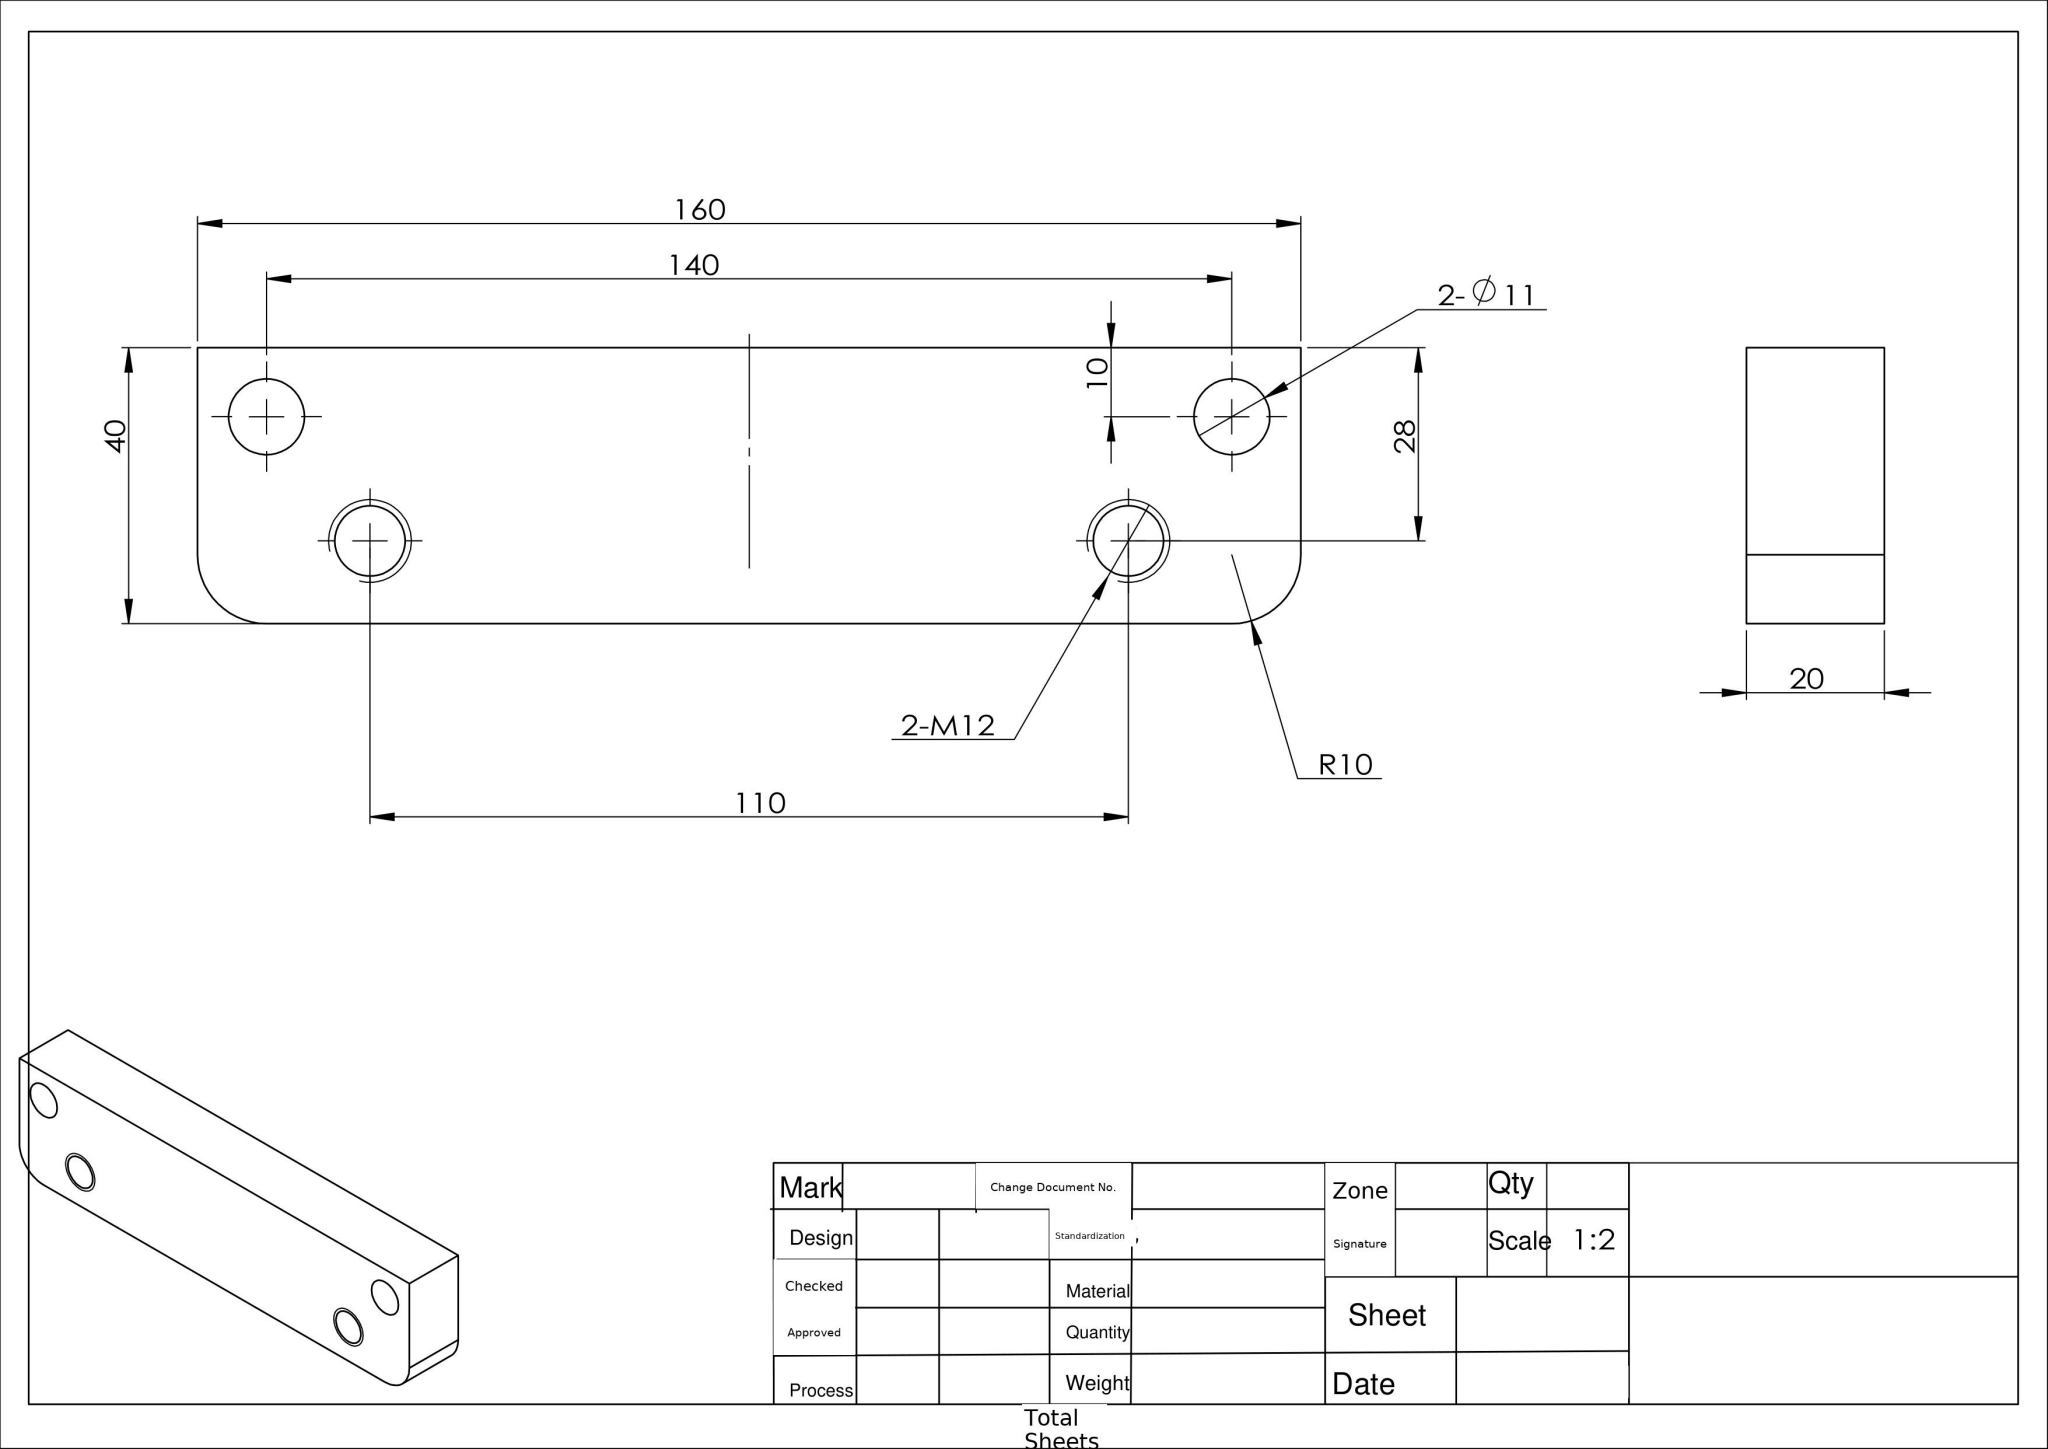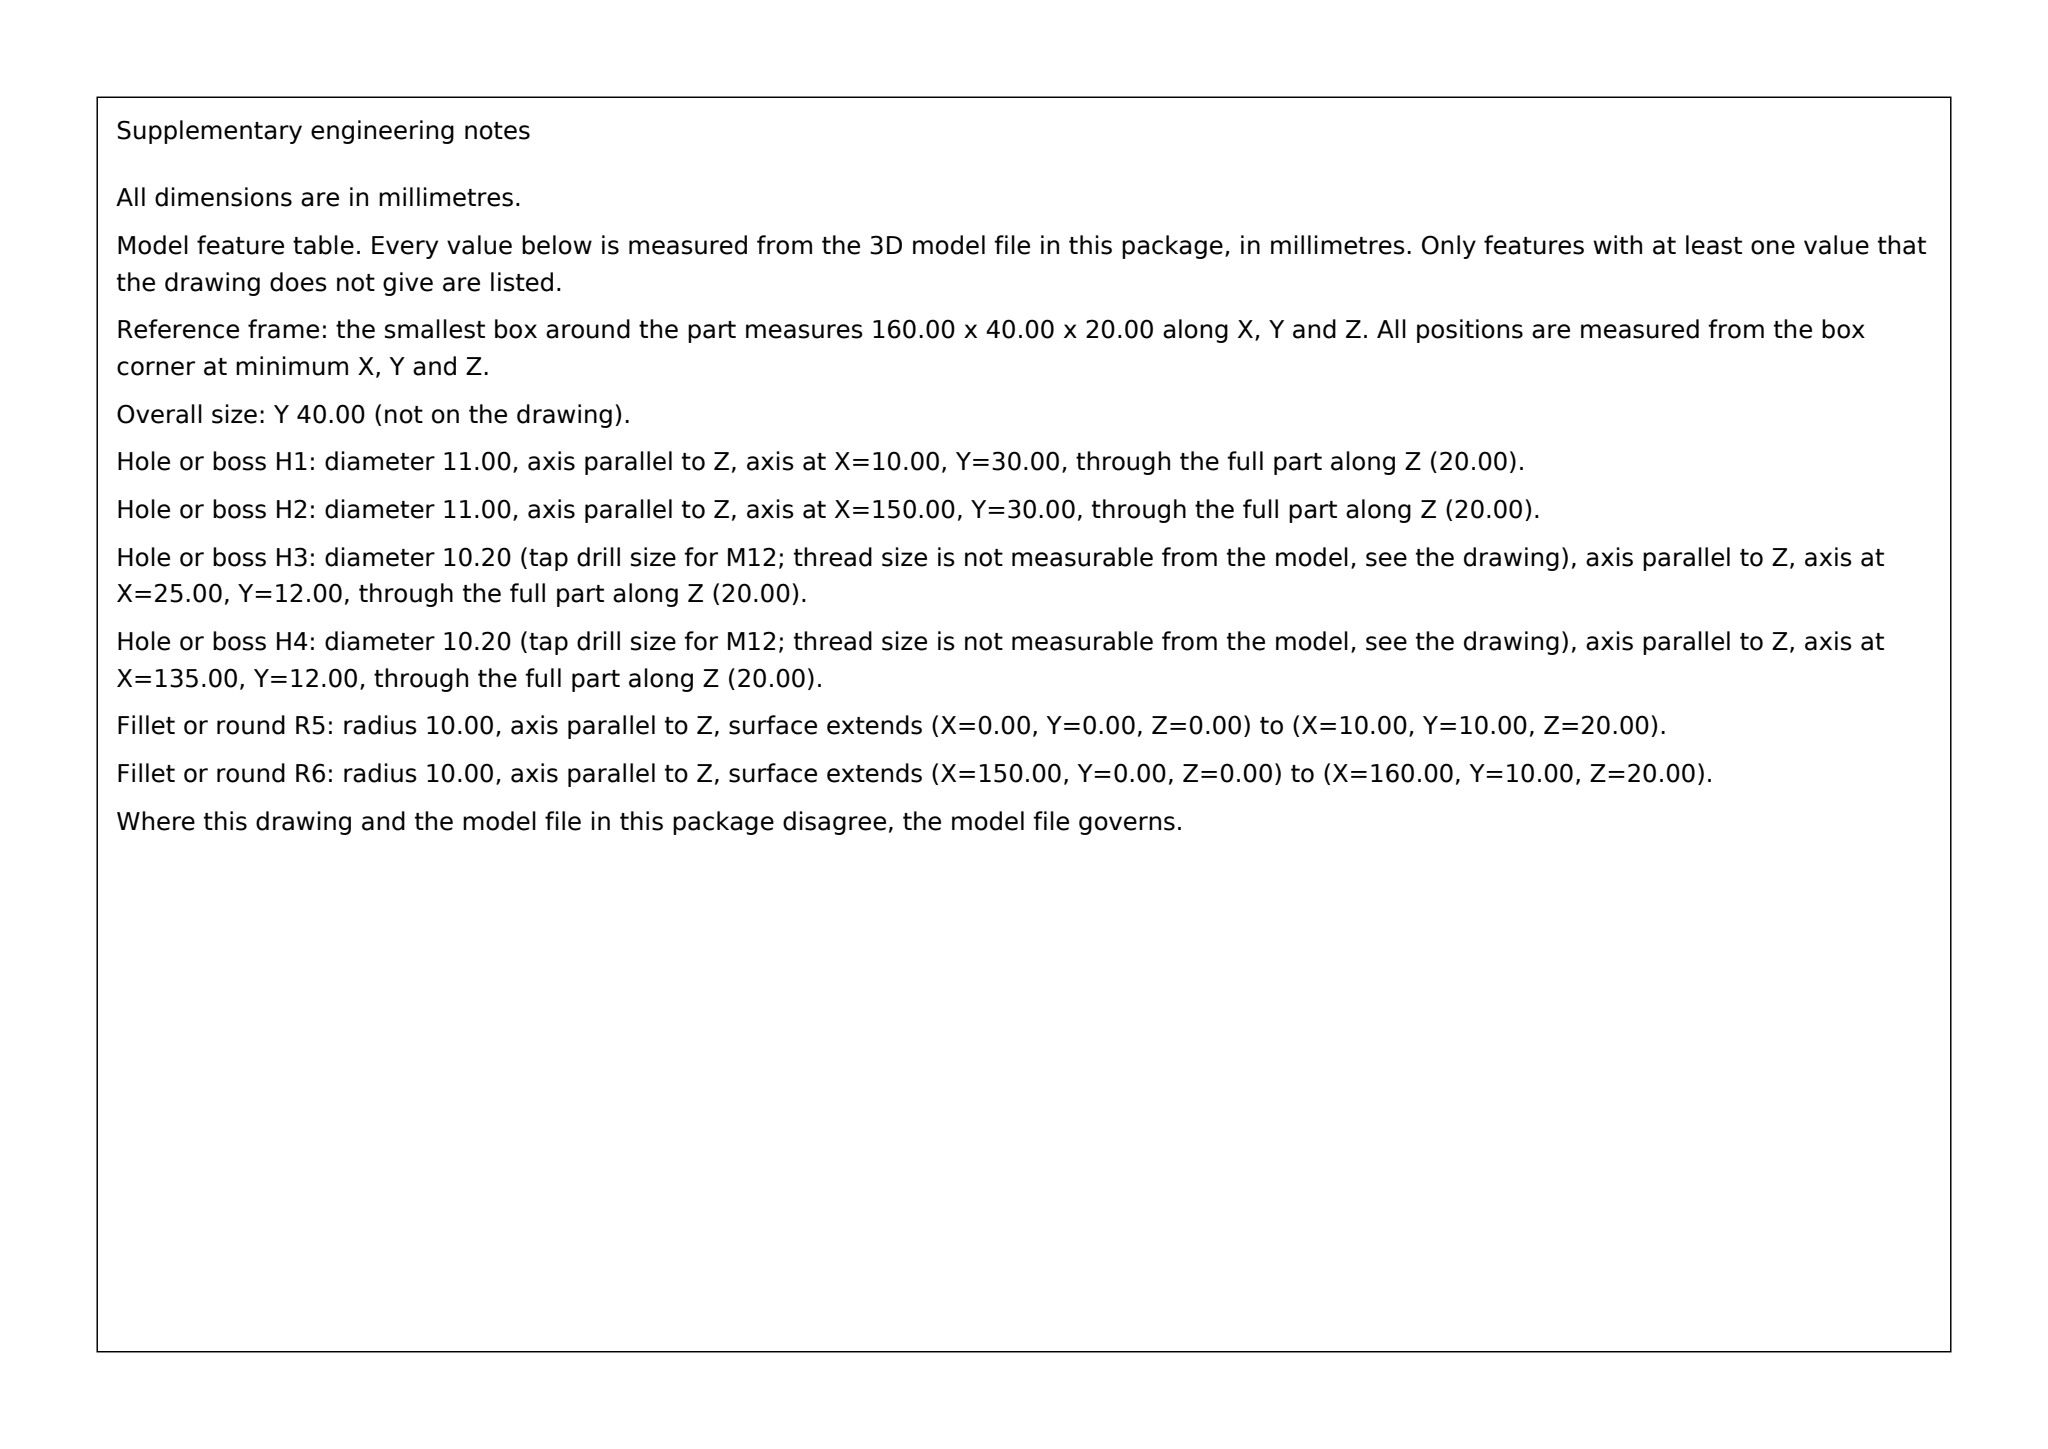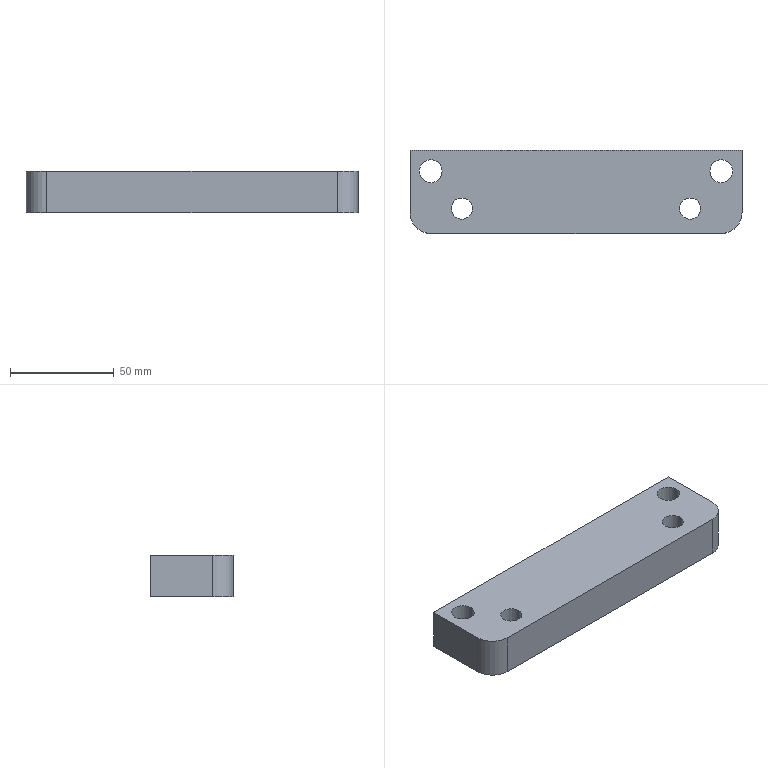Part | SolidWorks | 1 solid | 16 faces | box 160 x 40 x 20 mm | volume 120072 mm3 | cylinder 10 | plane 6 | commonest cylinder face diameters 10.2 x4 11 x4 20 x2
build123d program:
from build123d import *

# Parameters (mm, degrees)
SKETCH1_W              = 160
SKETCH1_H              = 40
BOSS_EXTRUDE1_DEPTH    = 20
SKETCH2_R              = 5.5
CUT_EXTRUDE1_DEPTH     = 20
M12_TAPPED_HOLE1_D     = 10.2
M12_TAPPED_HOLE1_DEPTH = 32.75
M12_TAPPED_HOLE1_TIP   = 3.064
FILLET1_R              = 10


with BuildPart() as part:
    # Sketch1 → Boss-Extrude1 (new body)
    with BuildSketch(Plane.XY):
        with Locations((80, 20)):
            Rectangle(SKETCH1_W, SKETCH1_H)
    extrude(amount=BOSS_EXTRUDE1_DEPTH)

    # Sketch2 → Cut-Extrude1 (cut)
    with BuildSketch(Plane.XY.offset(20)):
        with Locations((10, 30)):
            Circle(SKETCH2_R)
        with Locations((150, 30)):
            Circle(SKETCH2_R)
    extrude(amount=-CUT_EXTRUDE1_DEPTH, mode=Mode.SUBTRACT)

    # M12 Tapped Hole1
    with Locations(Plane.XY.offset(20)):
        with Locations((25, 12), (135, 12)):
            Hole(M12_TAPPED_HOLE1_D / 2, depth=M12_TAPPED_HOLE1_DEPTH)
            with Locations((0, 0, -(M12_TAPPED_HOLE1_DEPTH + M12_TAPPED_HOLE1_TIP / 2))):  # 118° drill point
                Cone(0, M12_TAPPED_HOLE1_D / 2, M12_TAPPED_HOLE1_TIP, mode=Mode.SUBTRACT)

    # Fillet1
    fillet1_edges = [part.edges().sort_by_distance(p)[0] for p in [
        (160, 0, 10),
        (0, 0, 10),
    ]]
    fillet(fillet1_edges, radius=FILLET1_R)


solid = part.part
STEP:
#1=CARTESIAN_POINT('',(30.1,12.,0.));
#2=VERTEX_POINT('',#1);
#3=CARTESIAN_POINT('',(19.9,12.,0.));
#4=VERTEX_POINT('',#3);
#5=CARTESIAN_POINT('',(25.,12.,0.));
#6=DIRECTION('',(0.,0.,-1.));
#7=DIRECTION('',(-1.,0.,0.));
#8=AXIS2_PLACEMENT_3D('',#5,#6,#7);
#9=CIRCLE('',#8,5.1);
#10=EDGE_CURVE('',#2,#4,#9,.T.);
#11=ORIENTED_EDGE('',*,*,#10,.T.);
#12=CARTESIAN_POINT('',(19.9,12.,20.));
#13=VERTEX_POINT('',#12);
#14=CARTESIAN_POINT('',(19.9,12.,20.));
#15=DIRECTION('',(0.,0.,1.));
#16=VECTOR('',#15,1000.);
#17=LINE('',#14,#16);
#18=EDGE_CURVE('',#4,#13,#17,.T.);
#19=ORIENTED_EDGE('',*,*,#18,.T.);
#20=CARTESIAN_POINT('',(30.1,12.,20.));
#21=VERTEX_POINT('',#20);
#22=CARTESIAN_POINT('',(25.,12.,20.));
#23=DIRECTION('',(0.,0.,1.));
#24=DIRECTION('',(1.,0.,0.));
#25=AXIS2_PLACEMENT_3D('',#22,#23,#24);
#26=CIRCLE('',#25,5.1);
#27=EDGE_CURVE('',#13,#21,#26,.T.);
#28=ORIENTED_EDGE('',*,*,#27,.T.);
#29=CARTESIAN_POINT('',(30.1,12.,20.));
#30=DIRECTION('',(0.,0.,1.));
#31=VECTOR('',#30,1000.);
#32=LINE('',#29,#31);
#33=EDGE_CURVE('',#2,#21,#32,.T.);
#34=ORIENTED_EDGE('',*,*,#33,.F.);
#35=EDGE_LOOP('',(#11,#19,#28,#34));
#36=FACE_OUTER_BOUND('',#35,.T.);
#37=CARTESIAN_POINT('',(25.,12.,20.));
#38=DIRECTION('',(0.,0.,1.));
#39=DIRECTION('',(1.,0.,0.));
#40=AXIS2_PLACEMENT_3D('',#37,#38,#39);
#41=CYLINDRICAL_SURFACE('',#40,5.1);
#42=ADVANCED_FACE('',(#36),#41,.F.);
#43=CARTESIAN_POINT('',(140.1,12.,0.));
#44=VERTEX_POINT('',#43);
#45=CARTESIAN_POINT('',(129.9,12.,0.));
#46=VERTEX_POINT('',#45);
#47=CARTESIAN_POINT('',(135.,12.,0.));
#48=DIRECTION('',(0.,0.,-1.));
#49=DIRECTION('',(-1.,0.,0.));
#50=AXIS2_PLACEMENT_3D('',#47,#48,#49);
#51=CIRCLE('',#50,5.1);
#52=EDGE_CURVE('',#44,#46,#51,.T.);
#53=ORIENTED_EDGE('',*,*,#52,.T.);
#54=CARTESIAN_POINT('',(129.9,12.,20.));
#55=VERTEX_POINT('',#54);
#56=CARTESIAN_POINT('',(129.9,12.,20.));
#57=DIRECTION('',(0.,0.,1.));
#58=VECTOR('',#57,1000.);
#59=LINE('',#56,#58);
#60=EDGE_CURVE('',#46,#55,#59,.T.);
#61=ORIENTED_EDGE('',*,*,#60,.T.);
#62=CARTESIAN_POINT('',(140.1,12.,20.));
#63=VERTEX_POINT('',#62);
#64=CARTESIAN_POINT('',(135.,12.,20.));
#65=DIRECTION('',(0.,0.,1.));
#66=DIRECTION('',(1.,0.,0.));
#67=AXIS2_PLACEMENT_3D('',#64,#65,#66);
#68=CIRCLE('',#67,5.1);
#69=EDGE_CURVE('',#55,#63,#68,.T.);
#70=ORIENTED_EDGE('',*,*,#69,.T.);
#71=CARTESIAN_POINT('',(140.1,12.,20.));
#72=DIRECTION('',(0.,0.,1.));
#73=VECTOR('',#72,1000.);
#74=LINE('',#71,#73);
#75=EDGE_CURVE('',#44,#63,#74,.T.);
#76=ORIENTED_EDGE('',*,*,#75,.F.);
#77=EDGE_LOOP('',(#53,#61,#70,#76));
#78=FACE_OUTER_BOUND('',#77,.T.);
#79=CARTESIAN_POINT('',(135.,12.,20.));
#80=DIRECTION('',(0.,0.,1.));
#81=DIRECTION('',(1.,0.,0.));
#82=AXIS2_PLACEMENT_3D('',#79,#80,#81);
#83=CYLINDRICAL_SURFACE('',#82,5.1);
#84=ADVANCED_FACE('',(#78),#83,.F.);
#85=CARTESIAN_POINT('',(144.5,30.,0.));
#86=VERTEX_POINT('',#85);
#87=CARTESIAN_POINT('',(155.5,30.,0.));
#88=VERTEX_POINT('',#87);
#89=CARTESIAN_POINT('',(150.,30.,0.));
#90=DIRECTION('',(0.,0.,1.));
#91=DIRECTION('',(1.,0.,0.));
#92=AXIS2_PLACEMENT_3D('',#89,#90,#91);
#93=CIRCLE('',#92,5.5);
#94=EDGE_CURVE('',#86,#88,#93,.T.);
#95=ORIENTED_EDGE('',*,*,#94,.F.);
#96=CARTESIAN_POINT('',(144.5,30.,20.));
#97=VERTEX_POINT('',#96);
#98=CARTESIAN_POINT('',(144.5,30.,0.));
#99=DIRECTION('',(0.,0.,1.));
#100=VECTOR('',#99,1000.);
#101=LINE('',#98,#100);
#102=EDGE_CURVE('',#86,#97,#101,.T.);
#103=ORIENTED_EDGE('',*,*,#102,.T.);
#104=CARTESIAN_POINT('',(155.5,30.,20.));
#105=VERTEX_POINT('',#104);
#106=CARTESIAN_POINT('',(150.,30.,20.));
#107=DIRECTION('',(0.,0.,1.));
#108=DIRECTION('',(1.,0.,0.));
#109=AXIS2_PLACEMENT_3D('',#106,#107,#108);
#110=CIRCLE('',#109,5.5);
#111=EDGE_CURVE('',#97,#105,#110,.T.);
#112=ORIENTED_EDGE('',*,*,#111,.T.);
#113=CARTESIAN_POINT('',(155.5,30.,0.));
#114=DIRECTION('',(0.,0.,1.));
#115=VECTOR('',#114,1000.);
#116=LINE('',#113,#115);
#117=EDGE_CURVE('',#88,#105,#116,.T.);
#118=ORIENTED_EDGE('',*,*,#117,.F.);
#119=EDGE_LOOP('',(#95,#103,#112,#118));
#120=FACE_OUTER_BOUND('',#119,.T.);
#121=CARTESIAN_POINT('',(150.,30.,0.));
#122=DIRECTION('',(0.,0.,1.));
#123=DIRECTION('',(1.,0.,0.));
#124=AXIS2_PLACEMENT_3D('',#121,#122,#123);
#125=CYLINDRICAL_SURFACE('',#124,5.5);
#126=ADVANCED_FACE('',(#120),#125,.F.);
#127=CARTESIAN_POINT('',(4.5,30.,0.));
#128=VERTEX_POINT('',#127);
#129=CARTESIAN_POINT('',(15.5,30.,0.));
#130=VERTEX_POINT('',#129);
#131=CARTESIAN_POINT('',(10.,30.,0.));
#132=DIRECTION('',(0.,0.,1.));
#133=DIRECTION('',(1.,0.,0.));
#134=AXIS2_PLACEMENT_3D('',#131,#132,#133);
#135=CIRCLE('',#134,5.5);
#136=EDGE_CURVE('',#128,#130,#135,.T.);
#137=ORIENTED_EDGE('',*,*,#136,.F.);
#138=CARTESIAN_POINT('',(4.5,30.,20.));
#139=VERTEX_POINT('',#138);
#140=CARTESIAN_POINT('',(4.5,30.,0.));
#141=DIRECTION('',(0.,0.,1.));
#142=VECTOR('',#141,1000.);
#143=LINE('',#140,#142);
#144=EDGE_CURVE('',#128,#139,#143,.T.);
#145=ORIENTED_EDGE('',*,*,#144,.T.);
#146=CARTESIAN_POINT('',(15.5,30.,20.));
#147=VERTEX_POINT('',#146);
#148=CARTESIAN_POINT('',(10.,30.,20.));
#149=DIRECTION('',(0.,0.,1.));
#150=DIRECTION('',(1.,0.,0.));
#151=AXIS2_PLACEMENT_3D('',#148,#149,#150);
#152=CIRCLE('',#151,5.5);
#153=EDGE_CURVE('',#139,#147,#152,.T.);
#154=ORIENTED_EDGE('',*,*,#153,.T.);
#155=CARTESIAN_POINT('',(15.5,30.,0.));
#156=DIRECTION('',(0.,0.,1.));
#157=VECTOR('',#156,1000.);
#158=LINE('',#155,#157);
#159=EDGE_CURVE('',#130,#147,#158,.T.);
#160=ORIENTED_EDGE('',*,*,#159,.F.);
#161=EDGE_LOOP('',(#137,#145,#154,#160));
#162=FACE_OUTER_BOUND('',#161,.T.);
#163=CARTESIAN_POINT('',(10.,30.,0.));
#164=DIRECTION('',(0.,0.,1.));
#165=DIRECTION('',(1.,0.,0.));
#166=AXIS2_PLACEMENT_3D('',#163,#164,#165);
#167=CYLINDRICAL_SURFACE('',#166,5.5);
#168=ADVANCED_FACE('',(#162),#167,.F.);
#169=CARTESIAN_POINT('',(0.,40.,0.));
#170=VERTEX_POINT('',#169);
#171=CARTESIAN_POINT('',(0.,10.,0.));
#172=VERTEX_POINT('',#171);
#173=CARTESIAN_POINT('',(0.,0.,0.));
#174=DIRECTION('',(0.,-1.,0.));
#175=VECTOR('',#174,1000.);
#176=LINE('',#173,#175);
#177=EDGE_CURVE('',#170,#172,#176,.T.);
#178=ORIENTED_EDGE('',*,*,#177,.T.);
#179=CARTESIAN_POINT('',(0.,10.,20.));
#180=VERTEX_POINT('',#179);
#181=CARTESIAN_POINT('',(0.,10.,20.));
#182=DIRECTION('',(0.,0.,1.));
#183=VECTOR('',#182,1000.);
#184=LINE('',#181,#183);
#185=EDGE_CURVE('',#172,#180,#184,.T.);
#186=ORIENTED_EDGE('',*,*,#185,.T.);
#187=CARTESIAN_POINT('',(0.,40.,20.));
#188=VERTEX_POINT('',#187);
#189=CARTESIAN_POINT('',(0.,0.,20.));
#190=DIRECTION('',(0.,-1.,0.));
#191=VECTOR('',#190,1000.);
#192=LINE('',#189,#191);
#193=EDGE_CURVE('',#188,#180,#192,.T.);
#194=ORIENTED_EDGE('',*,*,#193,.F.);
#195=CARTESIAN_POINT('',(0.,40.,20.));
#196=DIRECTION('',(0.,0.,-1.));
#197=VECTOR('',#196,1000.);
#198=LINE('',#195,#197);
#199=EDGE_CURVE('',#188,#170,#198,.T.);
#200=ORIENTED_EDGE('',*,*,#199,.T.);
#201=EDGE_LOOP('',(#178,#186,#194,#200));
#202=FACE_OUTER_BOUND('',#201,.T.);
#203=CARTESIAN_POINT('',(0.,0.,20.));
#204=DIRECTION('',(1.,0.,0.));
#205=DIRECTION('',(0.,0.,-1.));
#206=AXIS2_PLACEMENT_3D('',#203,#204,#205);
#207=PLANE('',#206);
#208=ADVANCED_FACE('',(#202),#207,.F.);
#209=CARTESIAN_POINT('',(10.,0.,20.));
#210=VERTEX_POINT('',#209);
#211=CARTESIAN_POINT('',(150.,0.,20.));
#212=VERTEX_POINT('',#211);
#213=CARTESIAN_POINT('',(0.,0.,20.));
#214=DIRECTION('',(1.,0.,0.));
#215=VECTOR('',#214,1000.);
#216=LINE('',#213,#215);
#217=EDGE_CURVE('',#210,#212,#216,.T.);
#218=ORIENTED_EDGE('',*,*,#217,.F.);
#219=CARTESIAN_POINT('',(10.,0.,0.));
#220=VERTEX_POINT('',#219);
#221=CARTESIAN_POINT('',(10.,0.,20.));
#222=DIRECTION('',(0.,0.,-1.));
#223=VECTOR('',#222,1000.);
#224=LINE('',#221,#223);
#225=EDGE_CURVE('',#210,#220,#224,.T.);
#226=ORIENTED_EDGE('',*,*,#225,.T.);
#227=CARTESIAN_POINT('',(150.,0.,0.));
#228=VERTEX_POINT('',#227);
#229=CARTESIAN_POINT('',(0.,0.,0.));
#230=DIRECTION('',(1.,0.,0.));
#231=VECTOR('',#230,1000.);
#232=LINE('',#229,#231);
#233=EDGE_CURVE('',#220,#228,#232,.T.);
#234=ORIENTED_EDGE('',*,*,#233,.T.);
#235=CARTESIAN_POINT('',(150.,0.,20.));
#236=DIRECTION('',(0.,0.,1.));
#237=VECTOR('',#236,1000.);
#238=LINE('',#235,#237);
#239=EDGE_CURVE('',#228,#212,#238,.T.);
#240=ORIENTED_EDGE('',*,*,#239,.T.);
#241=EDGE_LOOP('',(#218,#226,#234,#240));
#242=FACE_OUTER_BOUND('',#241,.T.);
#243=CARTESIAN_POINT('',(0.,0.,20.));
#244=DIRECTION('',(0.,1.,0.));
#245=DIRECTION('',(0.,0.,1.));
#246=AXIS2_PLACEMENT_3D('',#243,#244,#245);
#247=PLANE('',#246);
#248=ADVANCED_FACE('',(#242),#247,.F.);
#249=CARTESIAN_POINT('',(160.,10.,20.));
#250=VERTEX_POINT('',#249);
#251=CARTESIAN_POINT('',(160.,40.,20.));
#252=VERTEX_POINT('',#251);
#253=CARTESIAN_POINT('',(160.,0.,20.));
#254=DIRECTION('',(0.,1.,0.));
#255=VECTOR('',#254,1000.);
#256=LINE('',#253,#255);
#257=EDGE_CURVE('',#250,#252,#256,.T.);
#258=ORIENTED_EDGE('',*,*,#257,.F.);
#259=CARTESIAN_POINT('',(160.,10.,0.));
#260=VERTEX_POINT('',#259);
#261=CARTESIAN_POINT('',(160.,10.,20.));
#262=DIRECTION('',(0.,0.,-1.));
#263=VECTOR('',#262,1000.);
#264=LINE('',#261,#263);
#265=EDGE_CURVE('',#250,#260,#264,.T.);
#266=ORIENTED_EDGE('',*,*,#265,.T.);
#267=CARTESIAN_POINT('',(160.,40.,0.));
#268=VERTEX_POINT('',#267);
#269=CARTESIAN_POINT('',(160.,0.,0.));
#270=DIRECTION('',(0.,1.,0.));
#271=VECTOR('',#270,1000.);
#272=LINE('',#269,#271);
#273=EDGE_CURVE('',#260,#268,#272,.T.);
#274=ORIENTED_EDGE('',*,*,#273,.T.);
#275=CARTESIAN_POINT('',(160.,40.,20.));
#276=DIRECTION('',(0.,0.,-1.));
#277=VECTOR('',#276,1000.);
#278=LINE('',#275,#277);
#279=EDGE_CURVE('',#252,#268,#278,.T.);
#280=ORIENTED_EDGE('',*,*,#279,.F.);
#281=EDGE_LOOP('',(#258,#266,#274,#280));
#282=FACE_OUTER_BOUND('',#281,.T.);
#283=CARTESIAN_POINT('',(160.,0.,20.));
#284=DIRECTION('',(-1.,0.,0.));
#285=DIRECTION('',(0.,0.,1.));
#286=AXIS2_PLACEMENT_3D('',#283,#284,#285);
#287=PLANE('',#286);
#288=ADVANCED_FACE('',(#282),#287,.F.);
#289=CARTESIAN_POINT('',(0.,40.,0.));
#290=DIRECTION('',(-1.,0.,0.));
#291=VECTOR('',#290,1000.);
#292=LINE('',#289,#291);
#293=EDGE_CURVE('',#268,#170,#292,.T.);
#294=ORIENTED_EDGE('',*,*,#293,.T.);
#295=ORIENTED_EDGE('',*,*,#199,.F.);
#296=CARTESIAN_POINT('',(0.,40.,20.));
#297=DIRECTION('',(-1.,0.,0.));
#298=VECTOR('',#297,1000.);
#299=LINE('',#296,#298);
#300=EDGE_CURVE('',#252,#188,#299,.T.);
#301=ORIENTED_EDGE('',*,*,#300,.F.);
#302=ORIENTED_EDGE('',*,*,#279,.T.);
#303=EDGE_LOOP('',(#294,#295,#301,#302));
#304=FACE_OUTER_BOUND('',#303,.T.);
#305=CARTESIAN_POINT('',(0.,40.,20.));
#306=DIRECTION('',(0.,-1.,0.));
#307=DIRECTION('',(0.,0.,-1.));
#308=AXIS2_PLACEMENT_3D('',#305,#306,#307);
#309=PLANE('',#308);
#310=ADVANCED_FACE('',(#304),#309,.F.);
#311=CARTESIAN_POINT('',(25.,12.,20.));
#312=DIRECTION('',(0.,0.,1.));
#313=DIRECTION('',(1.,0.,0.));
#314=AXIS2_PLACEMENT_3D('',#311,#312,#313);
#315=CIRCLE('',#314,5.1);
#316=EDGE_CURVE('',#21,#13,#315,.T.);
#317=ORIENTED_EDGE('',*,*,#316,.F.);
#318=ORIENTED_EDGE('',*,*,#27,.F.);
#319=EDGE_LOOP('',(#317,#318));
#320=FACE_BOUND('',#319,.T.);
#321=CARTESIAN_POINT('',(135.,12.,20.));
#322=DIRECTION('',(0.,0.,1.));
#323=DIRECTION('',(1.,0.,0.));
#324=AXIS2_PLACEMENT_3D('',#321,#322,#323);
#325=CIRCLE('',#324,5.1);
#326=EDGE_CURVE('',#63,#55,#325,.T.);
#327=ORIENTED_EDGE('',*,*,#326,.F.);
#328=ORIENTED_EDGE('',*,*,#69,.F.);
#329=EDGE_LOOP('',(#327,#328));
#330=FACE_BOUND('',#329,.T.);
#331=CARTESIAN_POINT('',(150.,30.,20.));
#332=DIRECTION('',(0.,0.,1.));
#333=DIRECTION('',(1.,0.,0.));
#334=AXIS2_PLACEMENT_3D('',#331,#332,#333);
#335=CIRCLE('',#334,5.5);
#336=EDGE_CURVE('',#105,#97,#335,.T.);
#337=ORIENTED_EDGE('',*,*,#336,.F.);
#338=ORIENTED_EDGE('',*,*,#111,.F.);
#339=EDGE_LOOP('',(#337,#338));
#340=FACE_BOUND('',#339,.T.);
#341=CARTESIAN_POINT('',(10.,30.,20.));
#342=DIRECTION('',(0.,0.,1.));
#343=DIRECTION('',(1.,0.,0.));
#344=AXIS2_PLACEMENT_3D('',#341,#342,#343);
#345=CIRCLE('',#344,5.5);
#346=EDGE_CURVE('',#147,#139,#345,.T.);
#347=ORIENTED_EDGE('',*,*,#346,.F.);
#348=ORIENTED_EDGE('',*,*,#153,.F.);
#349=EDGE_LOOP('',(#347,#348));
#350=FACE_BOUND('',#349,.T.);
#351=ORIENTED_EDGE('',*,*,#193,.T.);
#352=CARTESIAN_POINT('',(10.,10.,20.));
#353=DIRECTION('',(0.,0.,1.));
#354=DIRECTION('',(-1.,0.,0.));
#355=AXIS2_PLACEMENT_3D('',#352,#353,#354);
#356=CIRCLE('',#355,10.);
#357=EDGE_CURVE('',#180,#210,#356,.T.);
#358=ORIENTED_EDGE('',*,*,#357,.T.);
#359=ORIENTED_EDGE('',*,*,#217,.T.);
#360=CARTESIAN_POINT('',(150.,10.,20.));
#361=DIRECTION('',(0.,0.,1.));
#362=DIRECTION('',(-1.,0.,0.));
#363=AXIS2_PLACEMENT_3D('',#360,#361,#362);
#364=CIRCLE('',#363,10.);
#365=EDGE_CURVE('',#212,#250,#364,.T.);
#366=ORIENTED_EDGE('',*,*,#365,.T.);
#367=ORIENTED_EDGE('',*,*,#257,.T.);
#368=ORIENTED_EDGE('',*,*,#300,.T.);
#369=EDGE_LOOP('',(#351,#358,#359,#366,#367,#368));
#370=FACE_OUTER_BOUND('',#369,.T.);
#371=CARTESIAN_POINT('',(0.,0.,20.));
#372=DIRECTION('',(0.,0.,-1.));
#373=DIRECTION('',(-1.,0.,0.));
#374=AXIS2_PLACEMENT_3D('',#371,#372,#373);
#375=PLANE('',#374);
#376=ADVANCED_FACE('',(#320,#330,#340,#350,#370),#375,.F.);
#377=ORIENTED_EDGE('',*,*,#10,.F.);
#378=CARTESIAN_POINT('',(25.,12.,0.));
#379=DIRECTION('',(0.,0.,-1.));
#380=DIRECTION('',(-1.,0.,0.));
#381=AXIS2_PLACEMENT_3D('',#378,#379,#380);
#382=CIRCLE('',#381,5.1);
#383=EDGE_CURVE('',#4,#2,#382,.T.);
#384=ORIENTED_EDGE('',*,*,#383,.F.);
#385=EDGE_LOOP('',(#377,#384));
#386=FACE_BOUND('',#385,.T.);
#387=ORIENTED_EDGE('',*,*,#52,.F.);
#388=CARTESIAN_POINT('',(135.,12.,0.));
#389=DIRECTION('',(0.,0.,-1.));
#390=DIRECTION('',(-1.,0.,0.));
#391=AXIS2_PLACEMENT_3D('',#388,#389,#390);
#392=CIRCLE('',#391,5.1);
#393=EDGE_CURVE('',#46,#44,#392,.T.);
#394=ORIENTED_EDGE('',*,*,#393,.F.);
#395=EDGE_LOOP('',(#387,#394));
#396=FACE_BOUND('',#395,.T.);
#397=CARTESIAN_POINT('',(150.,30.,0.));
#398=DIRECTION('',(0.,0.,1.));
#399=DIRECTION('',(1.,0.,0.));
#400=AXIS2_PLACEMENT_3D('',#397,#398,#399);
#401=CIRCLE('',#400,5.5);
#402=EDGE_CURVE('',#88,#86,#401,.T.);
#403=ORIENTED_EDGE('',*,*,#402,.T.);
#404=ORIENTED_EDGE('',*,*,#94,.T.);
#405=EDGE_LOOP('',(#403,#404));
#406=FACE_BOUND('',#405,.T.);
#407=CARTESIAN_POINT('',(10.,30.,0.));
#408=DIRECTION('',(0.,0.,1.));
#409=DIRECTION('',(1.,0.,0.));
#410=AXIS2_PLACEMENT_3D('',#407,#408,#409);
#411=CIRCLE('',#410,5.5);
#412=EDGE_CURVE('',#130,#128,#411,.T.);
#413=ORIENTED_EDGE('',*,*,#412,.T.);
#414=ORIENTED_EDGE('',*,*,#136,.T.);
#415=EDGE_LOOP('',(#413,#414));
#416=FACE_BOUND('',#415,.T.);
#417=ORIENTED_EDGE('',*,*,#233,.F.);
#418=CARTESIAN_POINT('',(10.,10.,0.));
#419=DIRECTION('',(0.,0.,-1.));
#420=DIRECTION('',(-1.,0.,0.));
#421=AXIS2_PLACEMENT_3D('',#418,#419,#420);
#422=CIRCLE('',#421,10.);
#423=EDGE_CURVE('',#220,#172,#422,.T.);
#424=ORIENTED_EDGE('',*,*,#423,.T.);
#425=ORIENTED_EDGE('',*,*,#177,.F.);
#426=ORIENTED_EDGE('',*,*,#293,.F.);
#427=ORIENTED_EDGE('',*,*,#273,.F.);
#428=CARTESIAN_POINT('',(150.,10.,0.));
#429=DIRECTION('',(0.,0.,-1.));
#430=DIRECTION('',(-1.,0.,0.));
#431=AXIS2_PLACEMENT_3D('',#428,#429,#430);
#432=CIRCLE('',#431,10.);
#433=EDGE_CURVE('',#260,#228,#432,.T.);
#434=ORIENTED_EDGE('',*,*,#433,.T.);
#435=EDGE_LOOP('',(#417,#424,#425,#426,#427,#434));
#436=FACE_OUTER_BOUND('',#435,.T.);
#437=CARTESIAN_POINT('',(0.,0.,0.));
#438=DIRECTION('',(0.,0.,-1.));
#439=DIRECTION('',(-1.,0.,0.));
#440=AXIS2_PLACEMENT_3D('',#437,#438,#439);
#441=PLANE('',#440);
#442=ADVANCED_FACE('',(#386,#396,#406,#416,#436),#441,.T.);
#443=ORIENTED_EDGE('',*,*,#144,.F.);
#444=ORIENTED_EDGE('',*,*,#412,.F.);
#445=ORIENTED_EDGE('',*,*,#159,.T.);
#446=ORIENTED_EDGE('',*,*,#346,.T.);
#447=EDGE_LOOP('',(#443,#444,#445,#446));
#448=FACE_OUTER_BOUND('',#447,.T.);
#449=CARTESIAN_POINT('',(10.,30.,0.));
#450=DIRECTION('',(0.,0.,1.));
#451=DIRECTION('',(1.,0.,0.));
#452=AXIS2_PLACEMENT_3D('',#449,#450,#451);
#453=CYLINDRICAL_SURFACE('',#452,5.5);
#454=ADVANCED_FACE('',(#448),#453,.F.);
#455=ORIENTED_EDGE('',*,*,#102,.F.);
#456=ORIENTED_EDGE('',*,*,#402,.F.);
#457=ORIENTED_EDGE('',*,*,#117,.T.);
#458=ORIENTED_EDGE('',*,*,#336,.T.);
#459=EDGE_LOOP('',(#455,#456,#457,#458));
#460=FACE_OUTER_BOUND('',#459,.T.);
#461=CARTESIAN_POINT('',(150.,30.,0.));
#462=DIRECTION('',(0.,0.,1.));
#463=DIRECTION('',(1.,0.,0.));
#464=AXIS2_PLACEMENT_3D('',#461,#462,#463);
#465=CYLINDRICAL_SURFACE('',#464,5.5);
#466=ADVANCED_FACE('',(#460),#465,.F.);
#467=ORIENTED_EDGE('',*,*,#60,.F.);
#468=ORIENTED_EDGE('',*,*,#393,.T.);
#469=ORIENTED_EDGE('',*,*,#75,.T.);
#470=ORIENTED_EDGE('',*,*,#326,.T.);
#471=EDGE_LOOP('',(#467,#468,#469,#470));
#472=FACE_OUTER_BOUND('',#471,.T.);
#473=CARTESIAN_POINT('',(135.,12.,20.));
#474=DIRECTION('',(0.,0.,1.));
#475=DIRECTION('',(1.,0.,0.));
#476=AXIS2_PLACEMENT_3D('',#473,#474,#475);
#477=CYLINDRICAL_SURFACE('',#476,5.1);
#478=ADVANCED_FACE('',(#472),#477,.F.);
#479=ORIENTED_EDGE('',*,*,#18,.F.);
#480=ORIENTED_EDGE('',*,*,#383,.T.);
#481=ORIENTED_EDGE('',*,*,#33,.T.);
#482=ORIENTED_EDGE('',*,*,#316,.T.);
#483=EDGE_LOOP('',(#479,#480,#481,#482));
#484=FACE_OUTER_BOUND('',#483,.T.);
#485=CARTESIAN_POINT('',(25.,12.,20.));
#486=DIRECTION('',(0.,0.,1.));
#487=DIRECTION('',(1.,0.,0.));
#488=AXIS2_PLACEMENT_3D('',#485,#486,#487);
#489=CYLINDRICAL_SURFACE('',#488,5.1);
#490=ADVANCED_FACE('',(#484),#489,.F.);
#491=ORIENTED_EDGE('',*,*,#357,.F.);
#492=ORIENTED_EDGE('',*,*,#185,.F.);
#493=ORIENTED_EDGE('',*,*,#423,.F.);
#494=ORIENTED_EDGE('',*,*,#225,.F.);
#495=EDGE_LOOP('',(#491,#492,#493,#494));
#496=FACE_OUTER_BOUND('',#495,.T.);
#497=CARTESIAN_POINT('',(10.,10.,20.));
#498=DIRECTION('',(0.,0.,-1.));
#499=DIRECTION('',(-1.,0.,0.));
#500=AXIS2_PLACEMENT_3D('',#497,#498,#499);
#501=CYLINDRICAL_SURFACE('',#500,10.);
#502=ADVANCED_FACE('',(#496),#501,.T.);
#503=ORIENTED_EDGE('',*,*,#365,.F.);
#504=ORIENTED_EDGE('',*,*,#239,.F.);
#505=ORIENTED_EDGE('',*,*,#433,.F.);
#506=ORIENTED_EDGE('',*,*,#265,.F.);
#507=EDGE_LOOP('',(#503,#504,#505,#506));
#508=FACE_OUTER_BOUND('',#507,.T.);
#509=CARTESIAN_POINT('',(150.,10.,20.));
#510=DIRECTION('',(0.,0.,-1.));
#511=DIRECTION('',(-1.,0.,0.));
#512=AXIS2_PLACEMENT_3D('',#509,#510,#511);
#513=CYLINDRICAL_SURFACE('',#512,10.);
#514=ADVANCED_FACE('',(#508),#513,.T.);
#515=CLOSED_SHELL('',(#42,#84,#126,#168,#208,#248,#288,#310,#376,#442,#454,#466,#478,#490,#502,#514));
#516=MANIFOLD_SOLID_BREP('',#515);
#517=CARTESIAN_POINT('',(0.,0.,0.));
#518=DIRECTION('',(0.,0.,1.));
#519=DIRECTION('',(1.,0.,0.));
#520=AXIS2_PLACEMENT_3D('',#517,#518,#519);
#521=(LENGTH_UNIT()NAMED_UNIT(*)SI_UNIT(.MILLI.,.METRE.));
#522=UNCERTAINTY_MEASURE_WITH_UNIT(LENGTH_MEASURE(0.00001),#521,'','');
#523=(NAMED_UNIT(*)PLANE_ANGLE_UNIT()SI_UNIT($,.RADIAN.));
#524=(NAMED_UNIT(*)SI_UNIT($,.STERADIAN.)SOLID_ANGLE_UNIT());
#525=(GEOMETRIC_REPRESENTATION_CONTEXT(3)GLOBAL_UNCERTAINTY_ASSIGNED_CONTEXT((#522))GLOBAL_UNIT_ASSIGNED_CONTEXT((#521,#523,#524))REPRESENTATION_CONTEXT('',''));
#526=ADVANCED_BREP_SHAPE_REPRESENTATION('',(#516,#520),#525);